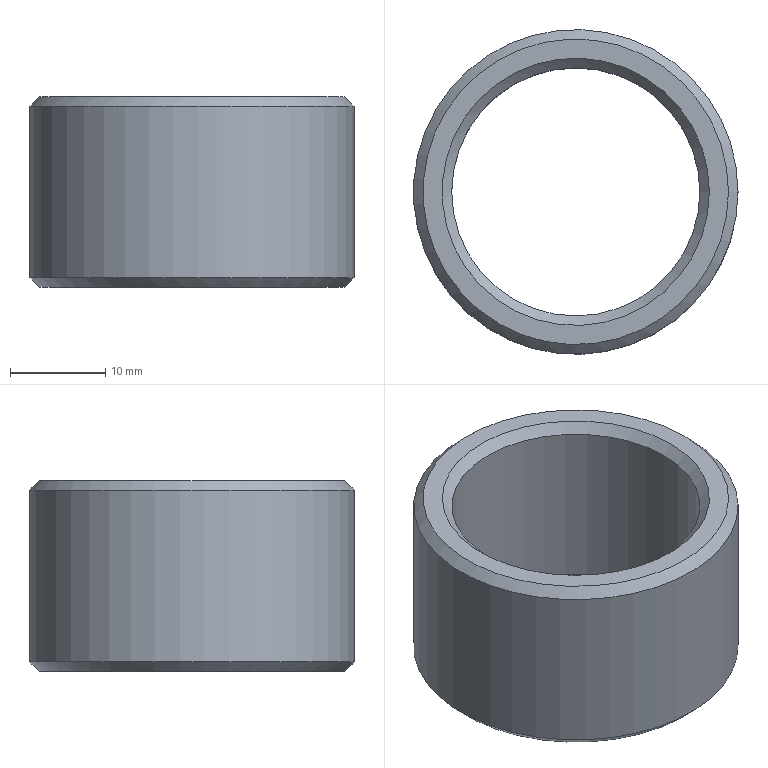Component | NX | BUSHING | 1 solid | 8 faces | box 34 x 34 x 20 mm | volume 7351 mm3 | cone 4 | cylinder 2 | plane 2 | commonest cylinder face diameters 34 x1 26 x1
STEP:
#1=CARTESIAN_POINT('',(0.,0.,0.));
#2=DIRECTION('',(0.,0.,1.));
#3=DIRECTION('',(1.,0.,0.));
#4=AXIS2_PLACEMENT_3D('',#1,#2,#3);
#5=CARTESIAN_POINT('',(49.,-0.,-159.));
#6=VERTEX_POINT('',#5);
#7=CARTESIAN_POINT('',(32.,-0.,-159.));
#8=DIRECTION('',(0.,0.,1.));
#9=DIRECTION('',(1.,0.,0.));
#10=AXIS2_PLACEMENT_3D('',#7,#8,#9);
#11=CIRCLE('',#10,17.);
#12=CARTESIAN_POINT('',(32.,-0.,-140.));
#13=DIRECTION('',(0.,0.,-1.));
#14=DIRECTION('',(-1.,0.,0.));
#15=AXIS2_PLACEMENT_3D('',#12,#13,#14);
#16=CYLINDRICAL_SURFACE('',#15,17.);
#17=CARTESIAN_POINT('',(9.425,19.));
#18=DIRECTION('',(-1.,0.));
#19=VECTOR('',#18,1.);
#20=LINE('',#17,#19);
#21=(GEOMETRIC_REPRESENTATION_CONTEXT(2)PARAMETRIC_REPRESENTATION_CONTEXT()REPRESENTATION_CONTEXT('',''));
#22=DEFINITIONAL_REPRESENTATION('',(#20),#21);
#23=PCURVE('',#16,#22);
#24=CARTESIAN_POINT('',(32.,-0.,-159.));
#25=DIRECTION('',(0.,0.,1.));
#26=DIRECTION('',(1.,0.,0.));
#27=AXIS2_PLACEMENT_3D('',#24,#25,#26);
#28=CONICAL_SURFACE('',#27,17.,0.7854);
#29=CARTESIAN_POINT('',(0.,0.));
#30=DIRECTION('',(1.,0.));
#31=VECTOR('',#30,1.);
#32=LINE('',#29,#31);
#33=(GEOMETRIC_REPRESENTATION_CONTEXT(2)PARAMETRIC_REPRESENTATION_CONTEXT()REPRESENTATION_CONTEXT('',''));
#34=DEFINITIONAL_REPRESENTATION('',(#32),#33);
#35=PCURVE('',#28,#34);
#36=SURFACE_CURVE('',#11,(#23,#35),.PCURVE_S1.);
#37=EDGE_CURVE('',#6,#6,#36,.T.);
#38=ORIENTED_EDGE('',*,*,#37,.T.);
#39=CARTESIAN_POINT('',(49.,-0.,-141.));
#40=VERTEX_POINT('',#39);
#41=CARTESIAN_POINT('',(49.,-0.,-141.));
#42=CARTESIAN_POINT('',(49.,-0.,-159.));
#43=B_SPLINE_CURVE_WITH_KNOTS('',1,(#41,#42),.UNSPECIFIED.,.F.,.F.,(2,2),(1.,19.),.PIECEWISE_BEZIER_KNOTS.);
#44=CARTESIAN_POINT('',(3.142,0.));
#45=DIRECTION('',(0.,1.));
#46=VECTOR('',#45,1.);
#47=LINE('',#44,#46);
#48=(GEOMETRIC_REPRESENTATION_CONTEXT(2)PARAMETRIC_REPRESENTATION_CONTEXT()REPRESENTATION_CONTEXT('',''));
#49=DEFINITIONAL_REPRESENTATION('',(#47),#48);
#50=PCURVE('',#16,#49);
#51=CARTESIAN_POINT('',(9.425,0.));
#52=DIRECTION('',(0.,1.));
#53=VECTOR('',#52,1.);
#54=LINE('',#51,#53);
#55=(GEOMETRIC_REPRESENTATION_CONTEXT(2)PARAMETRIC_REPRESENTATION_CONTEXT()REPRESENTATION_CONTEXT('',''));
#56=DEFINITIONAL_REPRESENTATION('',(#54),#55);
#57=PCURVE('',#16,#56);
#58=SEAM_CURVE('',#43,(#50,#57),.PCURVE_S1.);
#59=EDGE_CURVE('',#40,#6,#58,.T.);
#60=ORIENTED_EDGE('',*,*,#59,.F.);
#61=CARTESIAN_POINT('',(32.,-0.,-141.));
#62=DIRECTION('',(0.,0.,-1.));
#63=DIRECTION('',(1.,0.,0.));
#64=AXIS2_PLACEMENT_3D('',#61,#62,#63);
#65=CIRCLE('',#64,17.);
#66=CARTESIAN_POINT('',(3.142,1.));
#67=DIRECTION('',(1.,0.));
#68=VECTOR('',#67,1.);
#69=LINE('',#66,#68);
#70=(GEOMETRIC_REPRESENTATION_CONTEXT(2)PARAMETRIC_REPRESENTATION_CONTEXT()REPRESENTATION_CONTEXT('',''));
#71=DEFINITIONAL_REPRESENTATION('',(#69),#70);
#72=PCURVE('',#16,#71);
#73=CARTESIAN_POINT('',(32.,-0.,-140.));
#74=DIRECTION('',(0.,0.,-1.));
#75=DIRECTION('',(-1.,0.,0.));
#76=AXIS2_PLACEMENT_3D('',#73,#74,#75);
#77=CONICAL_SURFACE('',#76,16.,0.7854);
#78=CARTESIAN_POINT('',(3.142,1.));
#79=DIRECTION('',(1.,0.));
#80=VECTOR('',#79,1.);
#81=LINE('',#78,#80);
#82=(GEOMETRIC_REPRESENTATION_CONTEXT(2)PARAMETRIC_REPRESENTATION_CONTEXT()REPRESENTATION_CONTEXT('',''));
#83=DEFINITIONAL_REPRESENTATION('',(#81),#82);
#84=PCURVE('',#77,#83);
#85=SURFACE_CURVE('',#65,(#72,#84),.PCURVE_S1.);
#86=EDGE_CURVE('',#40,#40,#85,.T.);
#87=ORIENTED_EDGE('',*,*,#86,.T.);
#88=ORIENTED_EDGE('',*,*,#59,.T.);
#89=EDGE_LOOP('',(#38,#60,#87,#88));
#90=FACE_BOUND('',#89,.T.);
#91=ADVANCED_FACE('',(#90),#16,.T.);
#92=CARTESIAN_POINT('',(45.,-0.,-159.));
#93=VERTEX_POINT('',#92);
#94=CARTESIAN_POINT('',(32.,-0.,-159.));
#95=DIRECTION('',(0.,0.,-1.));
#96=DIRECTION('',(1.,0.,0.));
#97=AXIS2_PLACEMENT_3D('',#94,#95,#96);
#98=CIRCLE('',#97,13.);
#99=CARTESIAN_POINT('',(32.,-0.,-140.));
#100=DIRECTION('',(0.,0.,-1.));
#101=DIRECTION('',(-1.,0.,0.));
#102=AXIS2_PLACEMENT_3D('',#99,#100,#101);
#103=CYLINDRICAL_SURFACE('',#102,13.);
#104=CARTESIAN_POINT('',(3.142,19.));
#105=DIRECTION('',(1.,0.));
#106=VECTOR('',#105,1.);
#107=LINE('',#104,#106);
#108=(GEOMETRIC_REPRESENTATION_CONTEXT(2)PARAMETRIC_REPRESENTATION_CONTEXT()REPRESENTATION_CONTEXT('',''));
#109=DEFINITIONAL_REPRESENTATION('',(#107),#108);
#110=PCURVE('',#103,#109);
#111=CARTESIAN_POINT('',(32.,-0.,-160.));
#112=DIRECTION('',(0.,0.,-1.));
#113=DIRECTION('',(-1.,0.,0.));
#114=AXIS2_PLACEMENT_3D('',#111,#112,#113);
#115=CONICAL_SURFACE('',#114,14.,0.7854);
#116=CARTESIAN_POINT('',(3.142,-1.));
#117=DIRECTION('',(1.,0.));
#118=VECTOR('',#117,1.);
#119=LINE('',#116,#118);
#120=(GEOMETRIC_REPRESENTATION_CONTEXT(2)PARAMETRIC_REPRESENTATION_CONTEXT()REPRESENTATION_CONTEXT('',''));
#121=DEFINITIONAL_REPRESENTATION('',(#119),#120);
#122=PCURVE('',#115,#121);
#123=SURFACE_CURVE('',#98,(#110,#122),.PCURVE_S1.);
#124=EDGE_CURVE('',#93,#93,#123,.T.);
#125=ORIENTED_EDGE('',*,*,#124,.F.);
#126=CARTESIAN_POINT('',(45.,-0.,-141.));
#127=VERTEX_POINT('',#126);
#128=CARTESIAN_POINT('',(45.,-0.,-141.));
#129=CARTESIAN_POINT('',(45.,-0.,-159.));
#130=B_SPLINE_CURVE_WITH_KNOTS('',1,(#128,#129),.UNSPECIFIED.,.F.,.F.,(2,2),(1.,19.),.PIECEWISE_BEZIER_KNOTS.);
#131=CARTESIAN_POINT('',(3.142,0.));
#132=DIRECTION('',(0.,1.));
#133=VECTOR('',#132,1.);
#134=LINE('',#131,#133);
#135=(GEOMETRIC_REPRESENTATION_CONTEXT(2)PARAMETRIC_REPRESENTATION_CONTEXT()REPRESENTATION_CONTEXT('',''));
#136=DEFINITIONAL_REPRESENTATION('',(#134),#135);
#137=PCURVE('',#103,#136);
#138=CARTESIAN_POINT('',(9.425,0.));
#139=DIRECTION('',(0.,1.));
#140=VECTOR('',#139,1.);
#141=LINE('',#138,#140);
#142=(GEOMETRIC_REPRESENTATION_CONTEXT(2)PARAMETRIC_REPRESENTATION_CONTEXT()REPRESENTATION_CONTEXT('',''));
#143=DEFINITIONAL_REPRESENTATION('',(#141),#142);
#144=PCURVE('',#103,#143);
#145=SEAM_CURVE('',#130,(#137,#144),.PCURVE_S1.);
#146=EDGE_CURVE('',#127,#93,#145,.T.);
#147=ORIENTED_EDGE('',*,*,#146,.F.);
#148=CARTESIAN_POINT('',(32.,-0.,-141.));
#149=DIRECTION('',(0.,0.,1.));
#150=DIRECTION('',(1.,0.,0.));
#151=AXIS2_PLACEMENT_3D('',#148,#149,#150);
#152=CIRCLE('',#151,13.);
#153=CARTESIAN_POINT('',(9.425,1.));
#154=DIRECTION('',(-1.,0.));
#155=VECTOR('',#154,1.);
#156=LINE('',#153,#155);
#157=(GEOMETRIC_REPRESENTATION_CONTEXT(2)PARAMETRIC_REPRESENTATION_CONTEXT()REPRESENTATION_CONTEXT('',''));
#158=DEFINITIONAL_REPRESENTATION('',(#156),#157);
#159=PCURVE('',#103,#158);
#160=CARTESIAN_POINT('',(32.,-0.,-141.));
#161=DIRECTION('',(0.,0.,1.));
#162=DIRECTION('',(1.,0.,0.));
#163=AXIS2_PLACEMENT_3D('',#160,#161,#162);
#164=CONICAL_SURFACE('',#163,13.,0.7854);
#165=CARTESIAN_POINT('',(0.,0.));
#166=DIRECTION('',(1.,0.));
#167=VECTOR('',#166,1.);
#168=LINE('',#165,#167);
#169=(GEOMETRIC_REPRESENTATION_CONTEXT(2)PARAMETRIC_REPRESENTATION_CONTEXT()REPRESENTATION_CONTEXT('',''));
#170=DEFINITIONAL_REPRESENTATION('',(#168),#169);
#171=PCURVE('',#164,#170);
#172=SURFACE_CURVE('',#152,(#159,#171),.PCURVE_S1.);
#173=EDGE_CURVE('',#127,#127,#172,.T.);
#174=ORIENTED_EDGE('',*,*,#173,.F.);
#175=ORIENTED_EDGE('',*,*,#146,.T.);
#176=EDGE_LOOP('',(#125,#147,#174,#175));
#177=FACE_BOUND('',#176,.F.);
#178=ADVANCED_FACE('',(#177),#103,.F.);
#179=CARTESIAN_POINT('',(46.,-0.,-140.));
#180=VERTEX_POINT('',#179);
#181=CARTESIAN_POINT('',(32.,-0.,-140.));
#182=DIRECTION('',(0.,0.,-1.));
#183=DIRECTION('',(1.,0.,0.));
#184=AXIS2_PLACEMENT_3D('',#181,#182,#183);
#185=CIRCLE('',#184,14.);
#186=CARTESIAN_POINT('',(32.,-0.,-140.));
#187=DIRECTION('',(0.,0.,1.));
#188=DIRECTION('',(1.,0.,0.));
#189=AXIS2_PLACEMENT_3D('',#186,#187,#188);
#190=PLANE('',#189);
#191=CARTESIAN_POINT('',(14.,0.));
#192=CARTESIAN_POINT('',(14.,-24.249));
#193=CARTESIAN_POINT('',(-7.,-12.124));
#194=CARTESIAN_POINT('',(-28.,-0.));
#195=CARTESIAN_POINT('',(-7.,12.124));
#196=CARTESIAN_POINT('',(14.,24.249));
#197=CARTESIAN_POINT('',(14.,0.));
#198=(BOUNDED_CURVE()B_SPLINE_CURVE(2,(#191,#192,#193,#194,#195,#196,#197),.UNSPECIFIED.,.T.,.F.)B_SPLINE_CURVE_WITH_KNOTS((1,2,2,2,2,1),(-2.094,0.,2.094,4.189,6.283,8.378),.UNSPECIFIED.)CURVE()GEOMETRIC_REPRESENTATION_ITEM()RATIONAL_B_SPLINE_CURVE((1.,0.5,1.,0.5,1.,0.5,1.))REPRESENTATION_ITEM(''));
#199=(GEOMETRIC_REPRESENTATION_CONTEXT(2)PARAMETRIC_REPRESENTATION_CONTEXT()REPRESENTATION_CONTEXT('',''));
#200=DEFINITIONAL_REPRESENTATION('',(#198),#199);
#201=PCURVE('',#190,#200);
#202=CARTESIAN_POINT('',(6.283,1.));
#203=DIRECTION('',(-1.,0.));
#204=VECTOR('',#203,1.);
#205=LINE('',#202,#204);
#206=(GEOMETRIC_REPRESENTATION_CONTEXT(2)PARAMETRIC_REPRESENTATION_CONTEXT()REPRESENTATION_CONTEXT('',''));
#207=DEFINITIONAL_REPRESENTATION('',(#205),#206);
#208=PCURVE('',#164,#207);
#209=SURFACE_CURVE('',#185,(#201,#208),.PCURVE_S1.);
#210=EDGE_CURVE('',#180,#180,#209,.T.);
#211=ORIENTED_EDGE('',*,*,#210,.T.);
#212=EDGE_LOOP('',(#211));
#213=FACE_BOUND('',#212,.T.);
#214=CARTESIAN_POINT('',(48.,-0.,-140.));
#215=VERTEX_POINT('',#214);
#216=CARTESIAN_POINT('',(32.,-0.,-140.));
#217=DIRECTION('',(0.,0.,1.));
#218=DIRECTION('',(1.,0.,0.));
#219=AXIS2_PLACEMENT_3D('',#216,#217,#218);
#220=CIRCLE('',#219,16.);
#221=CARTESIAN_POINT('',(0.,0.));
#222=DIRECTION('',(1.,0.));
#223=AXIS2_PLACEMENT_2D('',#221,#222);
#224=CIRCLE('',#223,16.);
#225=(GEOMETRIC_REPRESENTATION_CONTEXT(2)PARAMETRIC_REPRESENTATION_CONTEXT()REPRESENTATION_CONTEXT('',''));
#226=DEFINITIONAL_REPRESENTATION('',(#224),#225);
#227=PCURVE('',#190,#226);
#228=CARTESIAN_POINT('',(9.425,0.));
#229=DIRECTION('',(-1.,0.));
#230=VECTOR('',#229,1.);
#231=LINE('',#228,#230);
#232=(GEOMETRIC_REPRESENTATION_CONTEXT(2)PARAMETRIC_REPRESENTATION_CONTEXT()REPRESENTATION_CONTEXT('',''));
#233=DEFINITIONAL_REPRESENTATION('',(#231),#232);
#234=PCURVE('',#77,#233);
#235=SURFACE_CURVE('',#220,(#227,#234),.PCURVE_S1.);
#236=EDGE_CURVE('',#215,#215,#235,.T.);
#237=ORIENTED_EDGE('',*,*,#236,.T.);
#238=EDGE_LOOP('',(#237));
#239=FACE_BOUND('',#238,.T.);
#240=ADVANCED_FACE('',(#213,#239),#190,.T.);
#241=CARTESIAN_POINT('',(46.,-0.,-160.));
#242=VERTEX_POINT('',#241);
#243=CARTESIAN_POINT('',(32.,-0.,-160.));
#244=DIRECTION('',(0.,0.,1.));
#245=DIRECTION('',(1.,0.,0.));
#246=AXIS2_PLACEMENT_3D('',#243,#244,#245);
#247=CIRCLE('',#246,14.);
#248=CARTESIAN_POINT('',(32.,-0.,-160.));
#249=DIRECTION('',(0.,0.,1.));
#250=DIRECTION('',(1.,0.,0.));
#251=AXIS2_PLACEMENT_3D('',#248,#249,#250);
#252=PLANE('',#251);
#253=CARTESIAN_POINT('',(0.,0.));
#254=DIRECTION('',(1.,0.));
#255=AXIS2_PLACEMENT_2D('',#253,#254);
#256=CIRCLE('',#255,14.);
#257=(GEOMETRIC_REPRESENTATION_CONTEXT(2)PARAMETRIC_REPRESENTATION_CONTEXT()REPRESENTATION_CONTEXT('',''));
#258=DEFINITIONAL_REPRESENTATION('',(#256),#257);
#259=PCURVE('',#252,#258);
#260=CARTESIAN_POINT('',(9.425,0.));
#261=DIRECTION('',(-1.,0.));
#262=VECTOR('',#261,1.);
#263=LINE('',#260,#262);
#264=(GEOMETRIC_REPRESENTATION_CONTEXT(2)PARAMETRIC_REPRESENTATION_CONTEXT()REPRESENTATION_CONTEXT('',''));
#265=DEFINITIONAL_REPRESENTATION('',(#263),#264);
#266=PCURVE('',#115,#265);
#267=SURFACE_CURVE('',#247,(#259,#266),.PCURVE_S1.);
#268=EDGE_CURVE('',#242,#242,#267,.T.);
#269=ORIENTED_EDGE('',*,*,#268,.T.);
#270=EDGE_LOOP('',(#269));
#271=FACE_BOUND('',#270,.T.);
#272=CARTESIAN_POINT('',(48.,-0.,-160.));
#273=VERTEX_POINT('',#272);
#274=CARTESIAN_POINT('',(32.,-0.,-160.));
#275=DIRECTION('',(0.,0.,-1.));
#276=DIRECTION('',(1.,0.,0.));
#277=AXIS2_PLACEMENT_3D('',#274,#275,#276);
#278=CIRCLE('',#277,16.);
#279=CARTESIAN_POINT('',(16.,0.));
#280=CARTESIAN_POINT('',(16.,-27.713));
#281=CARTESIAN_POINT('',(-8.,-13.856));
#282=CARTESIAN_POINT('',(-32.,-0.));
#283=CARTESIAN_POINT('',(-8.,13.856));
#284=CARTESIAN_POINT('',(16.,27.713));
#285=CARTESIAN_POINT('',(16.,0.));
#286=(BOUNDED_CURVE()B_SPLINE_CURVE(2,(#279,#280,#281,#282,#283,#284,#285),.UNSPECIFIED.,.T.,.F.)B_SPLINE_CURVE_WITH_KNOTS((1,2,2,2,2,1),(-2.094,0.,2.094,4.189,6.283,8.378),.UNSPECIFIED.)CURVE()GEOMETRIC_REPRESENTATION_ITEM()RATIONAL_B_SPLINE_CURVE((1.,0.5,1.,0.5,1.,0.5,1.))REPRESENTATION_ITEM(''));
#287=(GEOMETRIC_REPRESENTATION_CONTEXT(2)PARAMETRIC_REPRESENTATION_CONTEXT()REPRESENTATION_CONTEXT('',''));
#288=DEFINITIONAL_REPRESENTATION('',(#286),#287);
#289=PCURVE('',#252,#288);
#290=CARTESIAN_POINT('',(6.283,-1.));
#291=DIRECTION('',(-1.,0.));
#292=VECTOR('',#291,1.);
#293=LINE('',#290,#292);
#294=(GEOMETRIC_REPRESENTATION_CONTEXT(2)PARAMETRIC_REPRESENTATION_CONTEXT()REPRESENTATION_CONTEXT('',''));
#295=DEFINITIONAL_REPRESENTATION('',(#293),#294);
#296=PCURVE('',#28,#295);
#297=SURFACE_CURVE('',#278,(#289,#296),.PCURVE_S1.);
#298=EDGE_CURVE('',#273,#273,#297,.T.);
#299=ORIENTED_EDGE('',*,*,#298,.T.);
#300=EDGE_LOOP('',(#299));
#301=FACE_BOUND('',#300,.T.);
#302=ADVANCED_FACE('',(#271,#301),#252,.F.);
#303=ORIENTED_EDGE('',*,*,#124,.T.);
#304=CARTESIAN_POINT('',(45.,-0.,-159.));
#305=CARTESIAN_POINT('',(46.,-0.,-160.));
#306=B_SPLINE_CURVE_WITH_KNOTS('',1,(#304,#305),.UNSPECIFIED.,.F.,.F.,(2,2),(-1.414,0.),.PIECEWISE_BEZIER_KNOTS.);
#307=CARTESIAN_POINT('',(9.425,0.));
#308=DIRECTION('',(0.,1.));
#309=VECTOR('',#308,1.);
#310=LINE('',#307,#309);
#311=(GEOMETRIC_REPRESENTATION_CONTEXT(2)PARAMETRIC_REPRESENTATION_CONTEXT()REPRESENTATION_CONTEXT('',''));
#312=DEFINITIONAL_REPRESENTATION('',(#310),#311);
#313=PCURVE('',#115,#312);
#314=CARTESIAN_POINT('',(3.142,0.));
#315=DIRECTION('',(0.,1.));
#316=VECTOR('',#315,1.);
#317=LINE('',#314,#316);
#318=(GEOMETRIC_REPRESENTATION_CONTEXT(2)PARAMETRIC_REPRESENTATION_CONTEXT()REPRESENTATION_CONTEXT('',''));
#319=DEFINITIONAL_REPRESENTATION('',(#317),#318);
#320=PCURVE('',#115,#319);
#321=SEAM_CURVE('',#306,(#313,#320),.PCURVE_S1.);
#322=EDGE_CURVE('',#93,#242,#321,.T.);
#323=ORIENTED_EDGE('',*,*,#322,.T.);
#324=ORIENTED_EDGE('',*,*,#268,.T.);
#325=ORIENTED_EDGE('',*,*,#322,.F.);
#326=EDGE_LOOP('',(#303,#323,#324,#325));
#327=FACE_BOUND('',#326,.F.);
#328=ADVANCED_FACE('',(#327),#115,.F.);
#329=ORIENTED_EDGE('',*,*,#298,.F.);
#330=CARTESIAN_POINT('',(48.,-0.,-160.));
#331=CARTESIAN_POINT('',(49.,-0.,-159.));
#332=B_SPLINE_CURVE_WITH_KNOTS('',1,(#330,#331),.UNSPECIFIED.,.F.,.F.,(2,2),(-1.414,0.),.PIECEWISE_BEZIER_KNOTS.);
#333=CARTESIAN_POINT('',(6.283,0.));
#334=DIRECTION('',(0.,1.));
#335=VECTOR('',#334,1.);
#336=LINE('',#333,#335);
#337=(GEOMETRIC_REPRESENTATION_CONTEXT(2)PARAMETRIC_REPRESENTATION_CONTEXT()REPRESENTATION_CONTEXT('',''));
#338=DEFINITIONAL_REPRESENTATION('',(#336),#337);
#339=PCURVE('',#28,#338);
#340=CARTESIAN_POINT('',(0.,0.));
#341=DIRECTION('',(0.,1.));
#342=VECTOR('',#341,1.);
#343=LINE('',#340,#342);
#344=(GEOMETRIC_REPRESENTATION_CONTEXT(2)PARAMETRIC_REPRESENTATION_CONTEXT()REPRESENTATION_CONTEXT('',''));
#345=DEFINITIONAL_REPRESENTATION('',(#343),#344);
#346=PCURVE('',#28,#345);
#347=SEAM_CURVE('',#332,(#339,#346),.PCURVE_S1.);
#348=EDGE_CURVE('',#273,#6,#347,.T.);
#349=ORIENTED_EDGE('',*,*,#348,.T.);
#350=ORIENTED_EDGE('',*,*,#37,.F.);
#351=ORIENTED_EDGE('',*,*,#348,.F.);
#352=EDGE_LOOP('',(#329,#349,#350,#351));
#353=FACE_BOUND('',#352,.T.);
#354=ADVANCED_FACE('',(#353),#28,.T.);
#355=ORIENTED_EDGE('',*,*,#210,.T.);
#356=CARTESIAN_POINT('',(45.,-0.,-141.));
#357=CARTESIAN_POINT('',(46.,-0.,-140.));
#358=B_SPLINE_CURVE_WITH_KNOTS('',1,(#356,#357),.UNSPECIFIED.,.F.,.F.,(2,2),(0.,1.414),.PIECEWISE_BEZIER_KNOTS.);
#359=CARTESIAN_POINT('',(0.,0.));
#360=DIRECTION('',(0.,1.));
#361=VECTOR('',#360,1.);
#362=LINE('',#359,#361);
#363=(GEOMETRIC_REPRESENTATION_CONTEXT(2)PARAMETRIC_REPRESENTATION_CONTEXT()REPRESENTATION_CONTEXT('',''));
#364=DEFINITIONAL_REPRESENTATION('',(#362),#363);
#365=PCURVE('',#164,#364);
#366=CARTESIAN_POINT('',(6.283,0.));
#367=DIRECTION('',(0.,1.));
#368=VECTOR('',#367,1.);
#369=LINE('',#366,#368);
#370=(GEOMETRIC_REPRESENTATION_CONTEXT(2)PARAMETRIC_REPRESENTATION_CONTEXT()REPRESENTATION_CONTEXT('',''));
#371=DEFINITIONAL_REPRESENTATION('',(#369),#370);
#372=PCURVE('',#164,#371);
#373=SEAM_CURVE('',#358,(#365,#372),.PCURVE_S1.);
#374=EDGE_CURVE('',#127,#180,#373,.T.);
#375=ORIENTED_EDGE('',*,*,#374,.F.);
#376=ORIENTED_EDGE('',*,*,#173,.T.);
#377=ORIENTED_EDGE('',*,*,#374,.T.);
#378=EDGE_LOOP('',(#355,#375,#376,#377));
#379=FACE_BOUND('',#378,.F.);
#380=ADVANCED_FACE('',(#379),#164,.F.);
#381=ORIENTED_EDGE('',*,*,#86,.F.);
#382=CARTESIAN_POINT('',(48.,-0.,-140.));
#383=CARTESIAN_POINT('',(49.,-0.,-141.));
#384=B_SPLINE_CURVE_WITH_KNOTS('',1,(#382,#383),.UNSPECIFIED.,.F.,.F.,(2,2),(0.,1.414),.PIECEWISE_BEZIER_KNOTS.);
#385=CARTESIAN_POINT('',(3.142,0.));
#386=DIRECTION('',(0.,1.));
#387=VECTOR('',#386,1.);
#388=LINE('',#385,#387);
#389=(GEOMETRIC_REPRESENTATION_CONTEXT(2)PARAMETRIC_REPRESENTATION_CONTEXT()REPRESENTATION_CONTEXT('',''));
#390=DEFINITIONAL_REPRESENTATION('',(#388),#389);
#391=PCURVE('',#77,#390);
#392=CARTESIAN_POINT('',(9.425,0.));
#393=DIRECTION('',(0.,1.));
#394=VECTOR('',#393,1.);
#395=LINE('',#392,#394);
#396=(GEOMETRIC_REPRESENTATION_CONTEXT(2)PARAMETRIC_REPRESENTATION_CONTEXT()REPRESENTATION_CONTEXT('',''));
#397=DEFINITIONAL_REPRESENTATION('',(#395),#396);
#398=PCURVE('',#77,#397);
#399=SEAM_CURVE('',#384,(#391,#398),.PCURVE_S1.);
#400=EDGE_CURVE('',#215,#40,#399,.T.);
#401=ORIENTED_EDGE('',*,*,#400,.F.);
#402=ORIENTED_EDGE('',*,*,#236,.F.);
#403=ORIENTED_EDGE('',*,*,#400,.T.);
#404=EDGE_LOOP('',(#381,#401,#402,#403));
#405=FACE_BOUND('',#404,.T.);
#406=ADVANCED_FACE('',(#405),#77,.T.);
#407=CLOSED_SHELL('',(#91,#178,#240,#302,#328,#354,#380,#406));
#408=MANIFOLD_SOLID_BREP('',#407);
#409=(LENGTH_UNIT()NAMED_UNIT(*)SI_UNIT(.MILLI.,.METRE.));
#410=UNCERTAINTY_MEASURE_WITH_UNIT(LENGTH_MEASURE(0.00001),#409,'','');
#411=(NAMED_UNIT(*)PLANE_ANGLE_UNIT()SI_UNIT($,.RADIAN.));
#412=(NAMED_UNIT(*)SI_UNIT($,.STERADIAN.)SOLID_ANGLE_UNIT());
#413=(GEOMETRIC_REPRESENTATION_CONTEXT(3)GLOBAL_UNCERTAINTY_ASSIGNED_CONTEXT((#410))GLOBAL_UNIT_ASSIGNED_CONTEXT((#409,#411,#412))REPRESENTATION_CONTEXT('',''));
#414=ADVANCED_BREP_SHAPE_REPRESENTATION('',(#4,#408),#413);